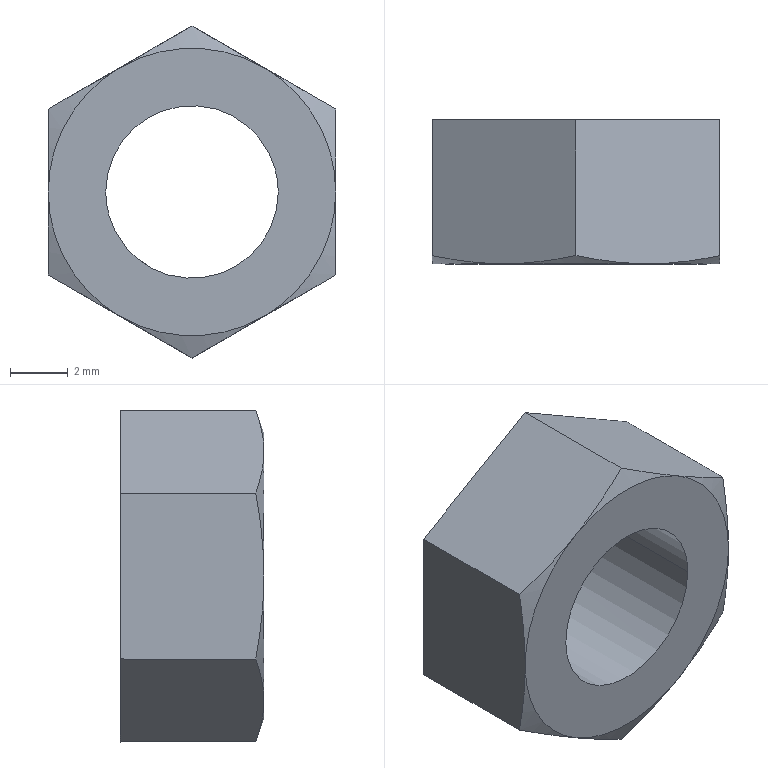Component | SolidWorks | TBK55-M6HexNut-1 | 1 solid | 16 faces | box 10 x 5 x 11.55 mm | volume 291 mm3 | plane 8 | cone 6 | cylinder 2 | commonest cylinder face diameters 6 x2
STEP:
#1=COLOUR_RGB('',0.7922,0.8196,0.9333);
#2=FILL_AREA_STYLE_COLOUR('',#1);
#3=FILL_AREA_STYLE('',(#2));
#4=SURFACE_STYLE_FILL_AREA(#3);
#5=SURFACE_SIDE_STYLE('',(#4));
#6=SURFACE_STYLE_USAGE(.BOTH.,#5);
#7=PRESENTATION_STYLE_ASSIGNMENT((#6));
#8=CARTESIAN_POINT('',(-4.908,1.968,7.539));
#9=VERTEX_POINT('',#8);
#10=CARTESIAN_POINT('',(-4.672,1.968,7.539));
#11=VERTEX_POINT('',#10);
#12=CARTESIAN_POINT('',(-4.908,1.968,7.539));
#13=CARTESIAN_POINT('',(-4.908,1.968,7.555));
#14=CARTESIAN_POINT('',(-4.905,1.968,7.57));
#15=CARTESIAN_POINT('',(-4.893,1.968,7.599));
#16=CARTESIAN_POINT('',(-4.884,1.968,7.612));
#17=CARTESIAN_POINT('',(-4.862,1.968,7.634));
#18=CARTESIAN_POINT('',(-4.849,1.968,7.643));
#19=CARTESIAN_POINT('',(-4.821,1.968,7.654));
#20=CARTESIAN_POINT('',(-4.805,1.968,7.657));
#21=CARTESIAN_POINT('',(-4.774,1.968,7.657));
#22=CARTESIAN_POINT('',(-4.759,1.968,7.654));
#23=CARTESIAN_POINT('',(-4.73,1.968,7.643));
#24=CARTESIAN_POINT('',(-4.717,1.968,7.634));
#25=CARTESIAN_POINT('',(-4.695,1.968,7.612));
#26=CARTESIAN_POINT('',(-4.687,1.968,7.599));
#27=CARTESIAN_POINT('',(-4.675,1.968,7.57));
#28=CARTESIAN_POINT('',(-4.672,1.968,7.555));
#29=CARTESIAN_POINT('',(-4.672,1.968,7.539));
#30=B_SPLINE_CURVE_WITH_KNOTS('',3,(#12,#13,#14,#15,#16,#17,#18,#19,#20,#21,#22,#23,#24,#25,#26,#27,#28,#29),.UNSPECIFIED.,.F.,.F.,(4,2,2,2,2,2,2,2,4),(0.,0.0625,0.125,0.1875,0.25,0.3125,0.375,0.4375,0.5),.UNSPECIFIED.);
#31=EDGE_CURVE('',#9,#11,#30,.T.);
#32=ORIENTED_EDGE('',*,*,#31,.F.);
#33=CARTESIAN_POINT('',(-4.908,2.165,7.539));
#34=VERTEX_POINT('',#33);
#35=CARTESIAN_POINT('',(-4.908,1.968,7.539));
#36=DIRECTION('',(0.,1.,0.));
#37=VECTOR('',#36,39.37);
#38=LINE('',#35,#37);
#39=EDGE_CURVE('',#9,#34,#38,.T.);
#40=ORIENTED_EDGE('',*,*,#39,.T.);
#41=CARTESIAN_POINT('',(-4.672,2.165,7.539));
#42=VERTEX_POINT('',#41);
#43=CARTESIAN_POINT('',(-4.908,2.165,7.539));
#44=CARTESIAN_POINT('',(-4.908,2.165,7.555));
#45=CARTESIAN_POINT('',(-4.905,2.165,7.57));
#46=CARTESIAN_POINT('',(-4.893,2.165,7.599));
#47=CARTESIAN_POINT('',(-4.884,2.165,7.612));
#48=CARTESIAN_POINT('',(-4.862,2.165,7.634));
#49=CARTESIAN_POINT('',(-4.849,2.165,7.643));
#50=CARTESIAN_POINT('',(-4.821,2.165,7.654));
#51=CARTESIAN_POINT('',(-4.805,2.165,7.657));
#52=CARTESIAN_POINT('',(-4.774,2.165,7.657));
#53=CARTESIAN_POINT('',(-4.759,2.165,7.654));
#54=CARTESIAN_POINT('',(-4.73,2.165,7.643));
#55=CARTESIAN_POINT('',(-4.717,2.165,7.634));
#56=CARTESIAN_POINT('',(-4.695,2.165,7.612));
#57=CARTESIAN_POINT('',(-4.687,2.165,7.599));
#58=CARTESIAN_POINT('',(-4.675,2.165,7.57));
#59=CARTESIAN_POINT('',(-4.672,2.165,7.555));
#60=CARTESIAN_POINT('',(-4.672,2.165,7.539));
#61=B_SPLINE_CURVE_WITH_KNOTS('',3,(#43,#44,#45,#46,#47,#48,#49,#50,#51,#52,#53,#54,#55,#56,#57,#58,#59,#60),.UNSPECIFIED.,.F.,.F.,(4,2,2,2,2,2,2,2,4),(0.5,0.5625,0.625,0.6875,0.75,0.8125,0.875,0.9375,1.),.UNSPECIFIED.);
#62=EDGE_CURVE('',#34,#42,#61,.T.);
#63=ORIENTED_EDGE('',*,*,#62,.T.);
#64=CARTESIAN_POINT('',(-4.672,1.968,7.539));
#65=DIRECTION('',(0.,1.,0.));
#66=VECTOR('',#65,39.37);
#67=LINE('',#64,#66);
#68=EDGE_CURVE('',#11,#42,#67,.T.);
#69=ORIENTED_EDGE('',*,*,#68,.F.);
#70=EDGE_LOOP('',(#32,#40,#63,#69));
#71=FACE_OUTER_BOUND('',#70,.T.);
#72=CARTESIAN_POINT('',(-4.79,1.968,7.539));
#73=DIRECTION('',(0.,1.,0.));
#74=DIRECTION('',(1.,0.,0.));
#75=AXIS2_PLACEMENT_3D('',#72,#73,#74);
#76=CYLINDRICAL_SURFACE('',#75,0.1181);
#77=ADVANCED_FACE('',(#71),#76,.F.);
#78=CARTESIAN_POINT('',(-4.672,2.165,7.539));
#79=CARTESIAN_POINT('',(-4.672,2.165,7.524));
#80=CARTESIAN_POINT('',(-4.675,2.165,7.508));
#81=CARTESIAN_POINT('',(-4.687,2.165,7.48));
#82=CARTESIAN_POINT('',(-4.695,2.165,7.467));
#83=CARTESIAN_POINT('',(-4.717,2.165,7.445));
#84=CARTESIAN_POINT('',(-4.73,2.165,7.436));
#85=CARTESIAN_POINT('',(-4.759,2.165,7.424));
#86=CARTESIAN_POINT('',(-4.774,2.165,7.421));
#87=CARTESIAN_POINT('',(-4.805,2.165,7.421));
#88=CARTESIAN_POINT('',(-4.821,2.165,7.424));
#89=CARTESIAN_POINT('',(-4.849,2.165,7.436));
#90=CARTESIAN_POINT('',(-4.862,2.165,7.445));
#91=CARTESIAN_POINT('',(-4.884,2.165,7.467));
#92=CARTESIAN_POINT('',(-4.893,2.165,7.48));
#93=CARTESIAN_POINT('',(-4.905,2.165,7.508));
#94=CARTESIAN_POINT('',(-4.908,2.165,7.524));
#95=CARTESIAN_POINT('',(-4.908,2.165,7.539));
#96=B_SPLINE_CURVE_WITH_KNOTS('',3,(#78,#79,#80,#81,#82,#83,#84,#85,#86,#87,#88,#89,#90,#91,#92,#93,#94,#95),.UNSPECIFIED.,.F.,.F.,(4,2,2,2,2,2,2,2,4),(0.,0.0625,0.125,0.1875,0.25,0.3125,0.375,0.4375,0.5),.UNSPECIFIED.);
#97=EDGE_CURVE('',#42,#34,#96,.T.);
#98=ORIENTED_EDGE('',*,*,#97,.F.);
#99=ORIENTED_EDGE('',*,*,#62,.F.);
#100=EDGE_LOOP('',(#98,#99));
#101=FACE_BOUND('',#100,.T.);
#102=CARTESIAN_POINT('',(-4.593,2.165,7.653));
#103=VERTEX_POINT('',#102);
#104=CARTESIAN_POINT('',(-4.593,2.165,7.426));
#105=VERTEX_POINT('',#104);
#106=CARTESIAN_POINT('',(-4.593,2.165,7.539));
#107=DIRECTION('',(0.,0.,-1.));
#108=VECTOR('',#107,39.37);
#109=LINE('',#106,#108);
#110=EDGE_CURVE('',#103,#105,#109,.T.);
#111=ORIENTED_EDGE('',*,*,#110,.T.);
#112=CARTESIAN_POINT('',(-4.79,2.165,7.312));
#113=VERTEX_POINT('',#112);
#114=CARTESIAN_POINT('',(-4.593,2.165,7.426));
#115=DIRECTION('',(-0.866,0.,-0.5));
#116=VECTOR('',#115,39.37);
#117=LINE('',#114,#116);
#118=EDGE_CURVE('',#105,#113,#117,.T.);
#119=ORIENTED_EDGE('',*,*,#118,.T.);
#120=CARTESIAN_POINT('',(-4.987,2.165,7.426));
#121=VERTEX_POINT('',#120);
#122=CARTESIAN_POINT('',(-4.79,2.165,7.312));
#123=DIRECTION('',(-0.866,0.,0.5));
#124=VECTOR('',#123,39.37);
#125=LINE('',#122,#124);
#126=EDGE_CURVE('',#113,#121,#125,.T.);
#127=ORIENTED_EDGE('',*,*,#126,.T.);
#128=CARTESIAN_POINT('',(-4.987,2.165,7.653));
#129=VERTEX_POINT('',#128);
#130=CARTESIAN_POINT('',(-4.987,2.165,7.539));
#131=DIRECTION('',(0.,0.,1.));
#132=VECTOR('',#131,39.37);
#133=LINE('',#130,#132);
#134=EDGE_CURVE('',#121,#129,#133,.T.);
#135=ORIENTED_EDGE('',*,*,#134,.T.);
#136=CARTESIAN_POINT('',(-4.79,2.165,7.767));
#137=VERTEX_POINT('',#136);
#138=CARTESIAN_POINT('',(-4.987,2.165,7.653));
#139=DIRECTION('',(0.866,0.,0.5));
#140=VECTOR('',#139,39.37);
#141=LINE('',#138,#140);
#142=EDGE_CURVE('',#129,#137,#141,.T.);
#143=ORIENTED_EDGE('',*,*,#142,.T.);
#144=CARTESIAN_POINT('',(-4.79,2.165,7.767));
#145=DIRECTION('',(0.866,0.,-0.5));
#146=VECTOR('',#145,39.37);
#147=LINE('',#144,#146);
#148=EDGE_CURVE('',#137,#103,#147,.T.);
#149=ORIENTED_EDGE('',*,*,#148,.T.);
#150=EDGE_LOOP('',(#111,#119,#127,#135,#143,#149));
#151=FACE_OUTER_BOUND('',#150,.T.);
#152=CARTESIAN_POINT('',(-4.79,2.165,7.539));
#153=DIRECTION('',(0.,1.,0.));
#154=DIRECTION('',(1.,0.,0.));
#155=AXIS2_PLACEMENT_3D('',#152,#153,#154);
#156=PLANE('',#155);
#157=ADVANCED_FACE('',(#101,#151),#156,.T.);
#158=CARTESIAN_POINT('',(-4.672,1.968,7.539));
#159=CARTESIAN_POINT('',(-4.672,1.968,7.524));
#160=CARTESIAN_POINT('',(-4.675,1.968,7.508));
#161=CARTESIAN_POINT('',(-4.687,1.968,7.48));
#162=CARTESIAN_POINT('',(-4.695,1.968,7.467));
#163=CARTESIAN_POINT('',(-4.717,1.968,7.445));
#164=CARTESIAN_POINT('',(-4.73,1.968,7.436));
#165=CARTESIAN_POINT('',(-4.759,1.968,7.424));
#166=CARTESIAN_POINT('',(-4.774,1.968,7.421));
#167=CARTESIAN_POINT('',(-4.805,1.968,7.421));
#168=CARTESIAN_POINT('',(-4.821,1.968,7.424));
#169=CARTESIAN_POINT('',(-4.849,1.968,7.436));
#170=CARTESIAN_POINT('',(-4.862,1.968,7.445));
#171=CARTESIAN_POINT('',(-4.884,1.968,7.467));
#172=CARTESIAN_POINT('',(-4.893,1.968,7.48));
#173=CARTESIAN_POINT('',(-4.905,1.968,7.508));
#174=CARTESIAN_POINT('',(-4.908,1.968,7.524));
#175=CARTESIAN_POINT('',(-4.908,1.968,7.539));
#176=B_SPLINE_CURVE_WITH_KNOTS('',3,(#158,#159,#160,#161,#162,#163,#164,#165,#166,#167,#168,#169,#170,#171,#172,#173,#174,#175),.UNSPECIFIED.,.F.,.F.,(4,2,2,2,2,2,2,2,4),(0.5,0.5625,0.625,0.6875,0.75,0.8125,0.875,0.9375,1.),.UNSPECIFIED.);
#177=EDGE_CURVE('',#11,#9,#176,.T.);
#178=ORIENTED_EDGE('',*,*,#177,.T.);
#179=ORIENTED_EDGE('',*,*,#31,.T.);
#180=EDGE_LOOP('',(#178,#179));
#181=FACE_BOUND('',#180,.T.);
#182=CARTESIAN_POINT('',(-4.888,1.968,7.71));
#183=VERTEX_POINT('',#182);
#184=CARTESIAN_POINT('',(-4.691,1.968,7.71));
#185=VERTEX_POINT('',#184);
#186=CARTESIAN_POINT('',(-4.79,1.968,7.539));
#187=DIRECTION('',(0.,1.,0.));
#188=DIRECTION('',(1.,0.,0.));
#189=AXIS2_PLACEMENT_3D('',#186,#187,#188);
#190=CIRCLE('',#189,0.1969);
#191=EDGE_CURVE('',#183,#185,#190,.T.);
#192=ORIENTED_EDGE('',*,*,#191,.F.);
#193=CARTESIAN_POINT('',(-4.987,1.968,7.539));
#194=VERTEX_POINT('',#193);
#195=CARTESIAN_POINT('',(-4.79,1.968,7.539));
#196=DIRECTION('',(0.,1.,0.));
#197=DIRECTION('',(1.,0.,0.));
#198=AXIS2_PLACEMENT_3D('',#195,#196,#197);
#199=CIRCLE('',#198,0.1969);
#200=EDGE_CURVE('',#194,#183,#199,.T.);
#201=ORIENTED_EDGE('',*,*,#200,.F.);
#202=CARTESIAN_POINT('',(-4.888,1.968,7.369));
#203=VERTEX_POINT('',#202);
#204=CARTESIAN_POINT('',(-4.79,1.968,7.539));
#205=DIRECTION('',(0.,1.,0.));
#206=DIRECTION('',(1.,0.,0.));
#207=AXIS2_PLACEMENT_3D('',#204,#205,#206);
#208=CIRCLE('',#207,0.1969);
#209=EDGE_CURVE('',#203,#194,#208,.T.);
#210=ORIENTED_EDGE('',*,*,#209,.F.);
#211=CARTESIAN_POINT('',(-4.691,1.968,7.369));
#212=VERTEX_POINT('',#211);
#213=CARTESIAN_POINT('',(-4.79,1.968,7.539));
#214=DIRECTION('',(0.,1.,0.));
#215=DIRECTION('',(1.,0.,0.));
#216=AXIS2_PLACEMENT_3D('',#213,#214,#215);
#217=CIRCLE('',#216,0.1969);
#218=EDGE_CURVE('',#212,#203,#217,.T.);
#219=ORIENTED_EDGE('',*,*,#218,.F.);
#220=CARTESIAN_POINT('',(-4.593,1.968,7.539));
#221=VERTEX_POINT('',#220);
#222=CARTESIAN_POINT('',(-4.79,1.968,7.539));
#223=DIRECTION('',(0.,1.,0.));
#224=DIRECTION('',(1.,0.,0.));
#225=AXIS2_PLACEMENT_3D('',#222,#223,#224);
#226=CIRCLE('',#225,0.1969);
#227=EDGE_CURVE('',#221,#212,#226,.T.);
#228=ORIENTED_EDGE('',*,*,#227,.F.);
#229=CARTESIAN_POINT('',(-4.79,1.968,7.539));
#230=DIRECTION('',(0.,1.,0.));
#231=DIRECTION('',(1.,0.,0.));
#232=AXIS2_PLACEMENT_3D('',#229,#230,#231);
#233=CIRCLE('',#232,0.1969);
#234=EDGE_CURVE('',#185,#221,#233,.T.);
#235=ORIENTED_EDGE('',*,*,#234,.F.);
#236=EDGE_LOOP('',(#192,#201,#210,#219,#228,#235));
#237=FACE_OUTER_BOUND('',#236,.T.);
#238=CARTESIAN_POINT('',(-4.79,1.968,7.539));
#239=DIRECTION('',(0.,1.,0.));
#240=DIRECTION('',(1.,0.,0.));
#241=AXIS2_PLACEMENT_3D('',#238,#239,#240);
#242=PLANE('',#241);
#243=ADVANCED_FACE('',(#181,#237),#242,.F.);
#244=CARTESIAN_POINT('',(-4.593,1.979,7.426));
#245=VERTEX_POINT('',#244);
#246=CARTESIAN_POINT('',(-4.691,1.968,7.369));
#247=CARTESIAN_POINT('',(-4.658,1.968,7.388));
#248=CARTESIAN_POINT('',(-4.626,1.973,7.407));
#249=CARTESIAN_POINT('',(-4.593,1.979,7.426));
#250=B_SPLINE_CURVE_WITH_KNOTS('',3,(#246,#247,#248,#249),.UNSPECIFIED.,.F.,.F.,(4,4),(0.,0.0029),.UNSPECIFIED.);
#251=EDGE_CURVE('',#212,#245,#250,.T.);
#252=ORIENTED_EDGE('',*,*,#251,.F.);
#253=CARTESIAN_POINT('',(-4.79,1.979,7.312));
#254=VERTEX_POINT('',#253);
#255=CARTESIAN_POINT('',(-4.79,1.979,7.312));
#256=CARTESIAN_POINT('',(-4.757,1.973,7.331));
#257=CARTESIAN_POINT('',(-4.725,1.968,7.35));
#258=CARTESIAN_POINT('',(-4.691,1.968,7.369));
#259=B_SPLINE_CURVE_WITH_KNOTS('',3,(#255,#256,#257,#258),.UNSPECIFIED.,.F.,.F.,(4,4),(0.,0.0029),.UNSPECIFIED.);
#260=EDGE_CURVE('',#254,#212,#259,.T.);
#261=ORIENTED_EDGE('',*,*,#260,.F.);
#262=CARTESIAN_POINT('',(-4.79,2.165,7.312));
#263=DIRECTION('',(0.,-1.,0.));
#264=VECTOR('',#263,39.37);
#265=LINE('',#262,#264);
#266=EDGE_CURVE('',#113,#254,#265,.T.);
#267=ORIENTED_EDGE('',*,*,#266,.F.);
#268=ORIENTED_EDGE('',*,*,#118,.F.);
#269=CARTESIAN_POINT('',(-4.593,2.165,7.426));
#270=DIRECTION('',(0.,1.,0.));
#271=VECTOR('',#270,39.37);
#272=LINE('',#269,#271);
#273=EDGE_CURVE('',#245,#105,#272,.T.);
#274=ORIENTED_EDGE('',*,*,#273,.F.);
#275=EDGE_LOOP('',(#252,#261,#267,#268,#274));
#276=FACE_OUTER_BOUND('',#275,.T.);
#277=CARTESIAN_POINT('',(-4.593,2.165,7.426));
#278=DIRECTION('',(-0.5,0.,0.866));
#279=DIRECTION('',(0.866,0.,0.5));
#280=AXIS2_PLACEMENT_3D('',#277,#278,#279);
#281=PLANE('',#280);
#282=ADVANCED_FACE('',(#276),#281,.F.);
#283=CARTESIAN_POINT('',(-4.593,1.979,7.653));
#284=VERTEX_POINT('',#283);
#285=CARTESIAN_POINT('',(-4.593,1.968,7.539));
#286=CARTESIAN_POINT('',(-4.593,1.968,7.578));
#287=CARTESIAN_POINT('',(-4.593,1.973,7.615));
#288=CARTESIAN_POINT('',(-4.593,1.979,7.653));
#289=B_SPLINE_CURVE_WITH_KNOTS('',3,(#285,#286,#287,#288),.UNSPECIFIED.,.F.,.F.,(4,4),(0.,0.0029),.UNSPECIFIED.);
#290=EDGE_CURVE('',#221,#284,#289,.T.);
#291=ORIENTED_EDGE('',*,*,#290,.F.);
#292=CARTESIAN_POINT('',(-4.593,1.979,7.426));
#293=CARTESIAN_POINT('',(-4.593,1.973,7.463));
#294=CARTESIAN_POINT('',(-4.593,1.968,7.501));
#295=CARTESIAN_POINT('',(-4.593,1.968,7.539));
#296=B_SPLINE_CURVE_WITH_KNOTS('',3,(#292,#293,#294,#295),.UNSPECIFIED.,.F.,.F.,(4,4),(0.,0.0029),.UNSPECIFIED.);
#297=EDGE_CURVE('',#245,#221,#296,.T.);
#298=ORIENTED_EDGE('',*,*,#297,.F.);
#299=ORIENTED_EDGE('',*,*,#273,.T.);
#300=ORIENTED_EDGE('',*,*,#110,.F.);
#301=CARTESIAN_POINT('',(-4.593,2.165,7.653));
#302=DIRECTION('',(0.,1.,0.));
#303=VECTOR('',#302,39.37);
#304=LINE('',#301,#303);
#305=EDGE_CURVE('',#284,#103,#304,.T.);
#306=ORIENTED_EDGE('',*,*,#305,.F.);
#307=EDGE_LOOP('',(#291,#298,#299,#300,#306));
#308=FACE_OUTER_BOUND('',#307,.T.);
#309=CARTESIAN_POINT('',(-4.593,2.165,7.653));
#310=DIRECTION('',(-1.,0.,0.));
#311=DIRECTION('',(0.,1.,0.));
#312=AXIS2_PLACEMENT_3D('',#309,#310,#311);
#313=PLANE('',#312);
#314=ADVANCED_FACE('',(#308),#313,.F.);
#315=CARTESIAN_POINT('',(-4.79,1.979,7.767));
#316=VERTEX_POINT('',#315);
#317=CARTESIAN_POINT('',(-4.691,1.968,7.71));
#318=CARTESIAN_POINT('',(-4.725,1.968,7.729));
#319=CARTESIAN_POINT('',(-4.757,1.973,7.748));
#320=CARTESIAN_POINT('',(-4.79,1.979,7.767));
#321=B_SPLINE_CURVE_WITH_KNOTS('',3,(#317,#318,#319,#320),.UNSPECIFIED.,.F.,.F.,(4,4),(0.,0.0029),.UNSPECIFIED.);
#322=EDGE_CURVE('',#185,#316,#321,.T.);
#323=ORIENTED_EDGE('',*,*,#322,.F.);
#324=CARTESIAN_POINT('',(-4.593,1.979,7.653));
#325=CARTESIAN_POINT('',(-4.626,1.973,7.672));
#326=CARTESIAN_POINT('',(-4.658,1.968,7.691));
#327=CARTESIAN_POINT('',(-4.691,1.968,7.71));
#328=B_SPLINE_CURVE_WITH_KNOTS('',3,(#324,#325,#326,#327),.UNSPECIFIED.,.F.,.F.,(4,4),(0.,0.0029),.UNSPECIFIED.);
#329=EDGE_CURVE('',#284,#185,#328,.T.);
#330=ORIENTED_EDGE('',*,*,#329,.F.);
#331=ORIENTED_EDGE('',*,*,#305,.T.);
#332=ORIENTED_EDGE('',*,*,#148,.F.);
#333=CARTESIAN_POINT('',(-4.79,2.165,7.767));
#334=DIRECTION('',(0.,1.,0.));
#335=VECTOR('',#334,39.37);
#336=LINE('',#333,#335);
#337=EDGE_CURVE('',#316,#137,#336,.T.);
#338=ORIENTED_EDGE('',*,*,#337,.F.);
#339=EDGE_LOOP('',(#323,#330,#331,#332,#338));
#340=FACE_OUTER_BOUND('',#339,.T.);
#341=CARTESIAN_POINT('',(-4.79,2.165,7.767));
#342=DIRECTION('',(-0.5,0.,-0.866));
#343=DIRECTION('',(-0.866,0.,0.5));
#344=AXIS2_PLACEMENT_3D('',#341,#342,#343);
#345=PLANE('',#344);
#346=ADVANCED_FACE('',(#340),#345,.F.);
#347=CARTESIAN_POINT('',(-4.987,1.979,7.653));
#348=VERTEX_POINT('',#347);
#349=CARTESIAN_POINT('',(-4.888,1.968,7.71));
#350=CARTESIAN_POINT('',(-4.921,1.968,7.691));
#351=CARTESIAN_POINT('',(-4.954,1.973,7.672));
#352=CARTESIAN_POINT('',(-4.987,1.979,7.653));
#353=B_SPLINE_CURVE_WITH_KNOTS('',3,(#349,#350,#351,#352),.UNSPECIFIED.,.F.,.F.,(4,4),(0.,0.0029),.UNSPECIFIED.);
#354=EDGE_CURVE('',#183,#348,#353,.T.);
#355=ORIENTED_EDGE('',*,*,#354,.F.);
#356=CARTESIAN_POINT('',(-4.79,1.979,7.767));
#357=CARTESIAN_POINT('',(-4.822,1.973,7.748));
#358=CARTESIAN_POINT('',(-4.855,1.968,7.729));
#359=CARTESIAN_POINT('',(-4.888,1.968,7.71));
#360=B_SPLINE_CURVE_WITH_KNOTS('',3,(#356,#357,#358,#359),.UNSPECIFIED.,.F.,.F.,(4,4),(0.,0.0029),.UNSPECIFIED.);
#361=EDGE_CURVE('',#316,#183,#360,.T.);
#362=ORIENTED_EDGE('',*,*,#361,.F.);
#363=ORIENTED_EDGE('',*,*,#337,.T.);
#364=ORIENTED_EDGE('',*,*,#142,.F.);
#365=CARTESIAN_POINT('',(-4.987,2.165,7.653));
#366=DIRECTION('',(0.,1.,0.));
#367=VECTOR('',#366,39.37);
#368=LINE('',#365,#367);
#369=EDGE_CURVE('',#348,#129,#368,.T.);
#370=ORIENTED_EDGE('',*,*,#369,.F.);
#371=EDGE_LOOP('',(#355,#362,#363,#364,#370));
#372=FACE_OUTER_BOUND('',#371,.T.);
#373=CARTESIAN_POINT('',(-4.987,2.165,7.653));
#374=DIRECTION('',(0.5,0.,-0.866));
#375=DIRECTION('',(-0.866,0.,-0.5));
#376=AXIS2_PLACEMENT_3D('',#373,#374,#375);
#377=PLANE('',#376);
#378=ADVANCED_FACE('',(#372),#377,.F.);
#379=CARTESIAN_POINT('',(-4.987,1.979,7.426));
#380=VERTEX_POINT('',#379);
#381=CARTESIAN_POINT('',(-4.987,1.968,7.539));
#382=CARTESIAN_POINT('',(-4.987,1.968,7.501));
#383=CARTESIAN_POINT('',(-4.987,1.973,7.463));
#384=CARTESIAN_POINT('',(-4.987,1.979,7.426));
#385=B_SPLINE_CURVE_WITH_KNOTS('',3,(#381,#382,#383,#384),.UNSPECIFIED.,.F.,.F.,(4,4),(0.,0.0029),.UNSPECIFIED.);
#386=EDGE_CURVE('',#194,#380,#385,.T.);
#387=ORIENTED_EDGE('',*,*,#386,.F.);
#388=CARTESIAN_POINT('',(-4.987,1.979,7.653));
#389=CARTESIAN_POINT('',(-4.987,1.973,7.615));
#390=CARTESIAN_POINT('',(-4.987,1.968,7.578));
#391=CARTESIAN_POINT('',(-4.987,1.968,7.539));
#392=B_SPLINE_CURVE_WITH_KNOTS('',3,(#388,#389,#390,#391),.UNSPECIFIED.,.F.,.F.,(4,4),(0.,0.0029),.UNSPECIFIED.);
#393=EDGE_CURVE('',#348,#194,#392,.T.);
#394=ORIENTED_EDGE('',*,*,#393,.F.);
#395=ORIENTED_EDGE('',*,*,#369,.T.);
#396=ORIENTED_EDGE('',*,*,#134,.F.);
#397=CARTESIAN_POINT('',(-4.987,2.165,7.426));
#398=DIRECTION('',(0.,1.,0.));
#399=VECTOR('',#398,39.37);
#400=LINE('',#397,#399);
#401=EDGE_CURVE('',#380,#121,#400,.T.);
#402=ORIENTED_EDGE('',*,*,#401,.F.);
#403=EDGE_LOOP('',(#387,#394,#395,#396,#402));
#404=FACE_OUTER_BOUND('',#403,.T.);
#405=CARTESIAN_POINT('',(-4.987,2.165,7.426));
#406=DIRECTION('',(1.,0.,0.));
#407=DIRECTION('',(0.,-1.,0.));
#408=AXIS2_PLACEMENT_3D('',#405,#406,#407);
#409=PLANE('',#408);
#410=ADVANCED_FACE('',(#404),#409,.F.);
#411=CARTESIAN_POINT('',(-4.888,1.968,7.369));
#412=CARTESIAN_POINT('',(-4.855,1.968,7.35));
#413=CARTESIAN_POINT('',(-4.822,1.973,7.331));
#414=CARTESIAN_POINT('',(-4.79,1.979,7.312));
#415=B_SPLINE_CURVE_WITH_KNOTS('',3,(#411,#412,#413,#414),.UNSPECIFIED.,.F.,.F.,(4,4),(0.,0.0029),.UNSPECIFIED.);
#416=EDGE_CURVE('',#203,#254,#415,.T.);
#417=ORIENTED_EDGE('',*,*,#416,.F.);
#418=CARTESIAN_POINT('',(-4.987,1.979,7.426));
#419=CARTESIAN_POINT('',(-4.954,1.973,7.407));
#420=CARTESIAN_POINT('',(-4.921,1.968,7.388));
#421=CARTESIAN_POINT('',(-4.888,1.968,7.369));
#422=B_SPLINE_CURVE_WITH_KNOTS('',3,(#418,#419,#420,#421),.UNSPECIFIED.,.F.,.F.,(4,4),(0.,0.0029),.UNSPECIFIED.);
#423=EDGE_CURVE('',#380,#203,#422,.T.);
#424=ORIENTED_EDGE('',*,*,#423,.F.);
#425=ORIENTED_EDGE('',*,*,#401,.T.);
#426=ORIENTED_EDGE('',*,*,#126,.F.);
#427=ORIENTED_EDGE('',*,*,#266,.T.);
#428=EDGE_LOOP('',(#417,#424,#425,#426,#427));
#429=FACE_OUTER_BOUND('',#428,.T.);
#430=CARTESIAN_POINT('',(-4.79,2.165,7.312));
#431=DIRECTION('',(0.5,0.,0.866));
#432=DIRECTION('',(0.866,0.,-0.5));
#433=AXIS2_PLACEMENT_3D('',#430,#431,#432);
#434=PLANE('',#433);
#435=ADVANCED_FACE('',(#429),#434,.F.);
#436=ORIENTED_EDGE('',*,*,#290,.T.);
#437=ORIENTED_EDGE('',*,*,#329,.T.);
#438=ORIENTED_EDGE('',*,*,#234,.T.);
#439=EDGE_LOOP('',(#436,#437,#438));
#440=FACE_OUTER_BOUND('',#439,.T.);
#441=CARTESIAN_POINT('',(-4.79,1.979,7.539));
#442=DIRECTION('',(0.,1.,0.));
#443=DIRECTION('',(1.,0.,0.));
#444=AXIS2_PLACEMENT_3D('',#441,#442,#443);
#445=CONICAL_SURFACE('',#444,0.2275,1.222);
#446=ADVANCED_FACE('',(#440),#445,.T.);
#447=ORIENTED_EDGE('',*,*,#322,.T.);
#448=ORIENTED_EDGE('',*,*,#361,.T.);
#449=ORIENTED_EDGE('',*,*,#191,.T.);
#450=EDGE_LOOP('',(#447,#448,#449));
#451=FACE_OUTER_BOUND('',#450,.T.);
#452=CARTESIAN_POINT('',(-4.79,1.979,7.539));
#453=DIRECTION('',(0.,1.,0.));
#454=DIRECTION('',(1.,0.,0.));
#455=AXIS2_PLACEMENT_3D('',#452,#453,#454);
#456=CONICAL_SURFACE('',#455,0.2275,1.222);
#457=ADVANCED_FACE('',(#451),#456,.T.);
#458=ORIENTED_EDGE('',*,*,#354,.T.);
#459=ORIENTED_EDGE('',*,*,#393,.T.);
#460=ORIENTED_EDGE('',*,*,#200,.T.);
#461=EDGE_LOOP('',(#458,#459,#460));
#462=FACE_OUTER_BOUND('',#461,.T.);
#463=CARTESIAN_POINT('',(-4.79,1.979,7.539));
#464=DIRECTION('',(0.,1.,0.));
#465=DIRECTION('',(1.,0.,0.));
#466=AXIS2_PLACEMENT_3D('',#463,#464,#465);
#467=CONICAL_SURFACE('',#466,0.2275,1.222);
#468=ADVANCED_FACE('',(#462),#467,.T.);
#469=ORIENTED_EDGE('',*,*,#386,.T.);
#470=ORIENTED_EDGE('',*,*,#423,.T.);
#471=ORIENTED_EDGE('',*,*,#209,.T.);
#472=EDGE_LOOP('',(#469,#470,#471));
#473=FACE_OUTER_BOUND('',#472,.T.);
#474=CARTESIAN_POINT('',(-4.79,1.979,7.539));
#475=DIRECTION('',(0.,1.,0.));
#476=DIRECTION('',(1.,0.,0.));
#477=AXIS2_PLACEMENT_3D('',#474,#475,#476);
#478=CONICAL_SURFACE('',#477,0.2275,1.222);
#479=ADVANCED_FACE('',(#473),#478,.T.);
#480=ORIENTED_EDGE('',*,*,#260,.T.);
#481=ORIENTED_EDGE('',*,*,#218,.T.);
#482=ORIENTED_EDGE('',*,*,#416,.T.);
#483=EDGE_LOOP('',(#480,#481,#482));
#484=FACE_OUTER_BOUND('',#483,.T.);
#485=CARTESIAN_POINT('',(-4.79,1.979,7.539));
#486=DIRECTION('',(0.,1.,0.));
#487=DIRECTION('',(1.,0.,0.));
#488=AXIS2_PLACEMENT_3D('',#485,#486,#487);
#489=CONICAL_SURFACE('',#488,0.2275,1.222);
#490=ADVANCED_FACE('',(#484),#489,.T.);
#491=ORIENTED_EDGE('',*,*,#251,.T.);
#492=ORIENTED_EDGE('',*,*,#297,.T.);
#493=ORIENTED_EDGE('',*,*,#227,.T.);
#494=EDGE_LOOP('',(#491,#492,#493));
#495=FACE_OUTER_BOUND('',#494,.T.);
#496=CARTESIAN_POINT('',(-4.79,1.979,7.539));
#497=DIRECTION('',(0.,1.,0.));
#498=DIRECTION('',(1.,0.,0.));
#499=AXIS2_PLACEMENT_3D('',#496,#497,#498);
#500=CONICAL_SURFACE('',#499,0.2275,1.222);
#501=ADVANCED_FACE('',(#495),#500,.T.);
#502=ORIENTED_EDGE('',*,*,#39,.F.);
#503=ORIENTED_EDGE('',*,*,#177,.F.);
#504=ORIENTED_EDGE('',*,*,#68,.T.);
#505=ORIENTED_EDGE('',*,*,#97,.T.);
#506=EDGE_LOOP('',(#502,#503,#504,#505));
#507=FACE_OUTER_BOUND('',#506,.T.);
#508=CARTESIAN_POINT('',(-4.79,1.968,7.539));
#509=DIRECTION('',(0.,1.,0.));
#510=DIRECTION('',(1.,0.,0.));
#511=AXIS2_PLACEMENT_3D('',#508,#509,#510);
#512=CYLINDRICAL_SURFACE('',#511,0.1181);
#513=ADVANCED_FACE('',(#507),#512,.F.);
#514=CLOSED_SHELL('',(#77,#157,#243,#282,#314,#346,#378,#410,#435,#446,#457,#468,#479,#490,#501,#513));
#515=MANIFOLD_SOLID_BREP('',#514);
#516=STYLED_ITEM('',(#7),#515);
#517=(LENGTH_UNIT()NAMED_UNIT(*)SI_UNIT($,.METRE.));
#518=LENGTH_MEASURE_WITH_UNIT(LENGTH_MEASURE(0.0254),#517);
#519=DIMENSIONAL_EXPONENTS(1.,0.,0.,0.,0.,0.,0.);
#520=(CONVERSION_BASED_UNIT('',#518)LENGTH_UNIT()NAMED_UNIT(#519));
#521=UNCERTAINTY_MEASURE_WITH_UNIT(LENGTH_MEASURE(0.00001),#520,'','');
#522=(NAMED_UNIT(*)PLANE_ANGLE_UNIT()SI_UNIT($,.RADIAN.));
#523=(NAMED_UNIT(*)SI_UNIT($,.STERADIAN.)SOLID_ANGLE_UNIT());
#524=(GEOMETRIC_REPRESENTATION_CONTEXT(3)GLOBAL_UNCERTAINTY_ASSIGNED_CONTEXT((#521))GLOBAL_UNIT_ASSIGNED_CONTEXT((#520,#522,#523))REPRESENTATION_CONTEXT('',''));
#525=MECHANICAL_DESIGN_GEOMETRIC_PRESENTATION_REPRESENTATION('',(#516),#524);
#526=PRESENTATION_LAYER_ASSIGNMENT('','',(#516));
#527=CARTESIAN_POINT('',(0.,0.,0.));
#528=DIRECTION('',(0.,0.,1.));
#529=DIRECTION('',(1.,0.,0.));
#530=AXIS2_PLACEMENT_3D('',#527,#528,#529);
#531=(LENGTH_UNIT()NAMED_UNIT(*)SI_UNIT($,.METRE.));
#532=LENGTH_MEASURE_WITH_UNIT(LENGTH_MEASURE(0.0254),#531);
#533=DIMENSIONAL_EXPONENTS(1.,0.,0.,0.,0.,0.,0.);
#534=(CONVERSION_BASED_UNIT('',#532)LENGTH_UNIT()NAMED_UNIT(#533));
#535=UNCERTAINTY_MEASURE_WITH_UNIT(LENGTH_MEASURE(0.00001),#534,'','');
#536=(NAMED_UNIT(*)PLANE_ANGLE_UNIT()SI_UNIT($,.RADIAN.));
#537=(NAMED_UNIT(*)SI_UNIT($,.STERADIAN.)SOLID_ANGLE_UNIT());
#538=(GEOMETRIC_REPRESENTATION_CONTEXT(3)GLOBAL_UNCERTAINTY_ASSIGNED_CONTEXT((#535))GLOBAL_UNIT_ASSIGNED_CONTEXT((#534,#536,#537))REPRESENTATION_CONTEXT('',''));
#539=ADVANCED_BREP_SHAPE_REPRESENTATION('',(#515,#530),#538);